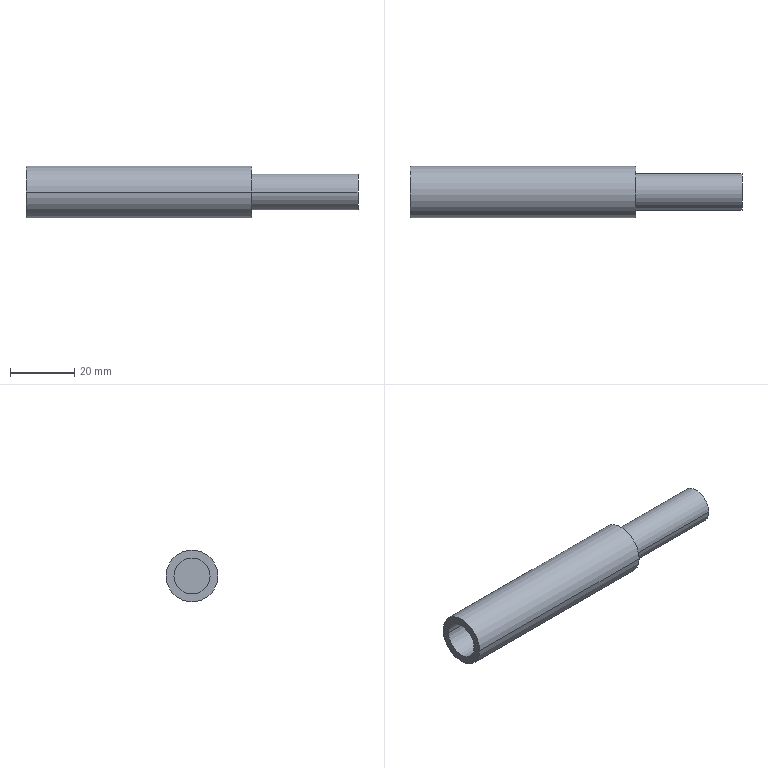Component | SolidWorks | MotorAxisHousing3-1 | 1 solid | 10 faces | box 103 x 16 x 16 mm | volume 12399 mm3 | cylinder 6 | plane 4 | commonest cylinder face diameters 11.2 x4 16 x2
build123d program:
from build123d import *

# Parameters (mm, degrees)
BOSS_EXTRUDE1_DEPTH      = 10
BOSS_EXTRUDE1_DEPTH_BACK = 43
SKETCH1_R                = 5.6
BOSS_EXTRUDE2_DEPTH      = 50
BOSS_EXTRUDE2_DEPTH_BACK = 20
SKETCH2_R                = 8
SKETCH2_R_2              = 5.6


with BuildPart() as part:
    # Sketch1 → Boss-Extrude1 (new, two sides: drawn at the far end of the back side and taken through both)
    with BuildSketch(Plane.XY.offset(-BOSS_EXTRUDE1_DEPTH_BACK)):
        with Locations((92, 0)):
            Circle(SKETCH1_R)
    extrude(amount=BOSS_EXTRUDE1_DEPTH + BOSS_EXTRUDE1_DEPTH_BACK)

    # Sketch2 → Boss-Extrude2 (add, two sides: drawn at the far end of the back side and taken through both)
    with BuildSketch(Plane.XY.offset(10).offset(-BOSS_EXTRUDE2_DEPTH_BACK)):
        with Locations((92, 0)):
            Circle(SKETCH2_R)
        with Locations((92, 0)):
            Circle(SKETCH2_R_2, mode=Mode.SUBTRACT)
    extrude(amount=BOSS_EXTRUDE2_DEPTH + BOSS_EXTRUDE2_DEPTH_BACK)


solid = part.part

# Placed as in the assembly
solid = solid.moved(Location((-500, 92, -92), (0, -90, 0)))
STEP:
#1=COLOUR_RGB('',0.7922,0.8196,0.9333);
#2=FILL_AREA_STYLE_COLOUR('',#1);
#3=FILL_AREA_STYLE('',(#2));
#4=SURFACE_STYLE_FILL_AREA(#3);
#5=SURFACE_SIDE_STYLE('',(#4));
#6=SURFACE_STYLE_USAGE(.BOTH.,#5);
#7=PRESENTATION_STYLE_ASSIGNMENT((#6));
#8=CARTESIAN_POINT('',(-20.079,3.402,0.));
#9=VERTEX_POINT('',#8);
#10=CARTESIAN_POINT('',(-20.079,3.843,0.));
#11=VERTEX_POINT('',#10);
#12=CARTESIAN_POINT('',(-20.079,3.622,0.));
#13=DIRECTION('',(-1.,0.,0.));
#14=DIRECTION('',(0.,1.,0.));
#15=AXIS2_PLACEMENT_3D('',#12,#13,#14);
#16=CIRCLE('',#15,0.2205);
#17=EDGE_CURVE('',#9,#11,#16,.T.);
#18=ORIENTED_EDGE('',*,*,#17,.F.);
#19=CARTESIAN_POINT('',(-22.047,3.402,0.));
#20=VERTEX_POINT('',#19);
#21=CARTESIAN_POINT('',(-19.291,3.402,0.));
#22=DIRECTION('',(-1.,0.,0.));
#23=VECTOR('',#22,39.37);
#24=LINE('',#21,#23);
#25=EDGE_CURVE('',#9,#20,#24,.T.);
#26=ORIENTED_EDGE('',*,*,#25,.T.);
#27=CARTESIAN_POINT('',(-22.047,3.843,0.));
#28=VERTEX_POINT('',#27);
#29=CARTESIAN_POINT('',(-22.047,3.622,0.));
#30=DIRECTION('',(-1.,0.,0.));
#31=DIRECTION('',(0.,1.,0.));
#32=AXIS2_PLACEMENT_3D('',#29,#30,#31);
#33=CIRCLE('',#32,0.2205);
#34=EDGE_CURVE('',#20,#28,#33,.T.);
#35=ORIENTED_EDGE('',*,*,#34,.T.);
#36=CARTESIAN_POINT('',(-19.291,3.843,0.));
#37=DIRECTION('',(-1.,0.,0.));
#38=VECTOR('',#37,39.37);
#39=LINE('',#36,#38);
#40=EDGE_CURVE('',#11,#28,#39,.T.);
#41=ORIENTED_EDGE('',*,*,#40,.F.);
#42=EDGE_LOOP('',(#18,#26,#35,#41));
#43=FACE_OUTER_BOUND('',#42,.T.);
#44=CARTESIAN_POINT('',(-19.291,3.622,0.));
#45=DIRECTION('',(-1.,0.,0.));
#46=DIRECTION('',(0.,1.,0.));
#47=AXIS2_PLACEMENT_3D('',#44,#45,#46);
#48=CYLINDRICAL_SURFACE('',#47,0.2205);
#49=ADVANCED_FACE('',(#43),#48,.F.);
#50=CARTESIAN_POINT('',(-19.291,3.937,0.));
#51=VERTEX_POINT('',#50);
#52=CARTESIAN_POINT('',(-19.291,3.307,0.));
#53=VERTEX_POINT('',#52);
#54=CARTESIAN_POINT('',(-19.291,3.622,0.));
#55=DIRECTION('',(-1.,0.,0.));
#56=DIRECTION('',(0.,1.,0.));
#57=AXIS2_PLACEMENT_3D('',#54,#55,#56);
#58=CIRCLE('',#57,0.315);
#59=EDGE_CURVE('',#51,#53,#58,.T.);
#60=ORIENTED_EDGE('',*,*,#59,.T.);
#61=CARTESIAN_POINT('',(-22.047,3.307,0.));
#62=VERTEX_POINT('',#61);
#63=CARTESIAN_POINT('',(-19.291,3.307,0.));
#64=DIRECTION('',(-1.,0.,0.));
#65=VECTOR('',#64,39.37);
#66=LINE('',#63,#65);
#67=EDGE_CURVE('',#53,#62,#66,.T.);
#68=ORIENTED_EDGE('',*,*,#67,.T.);
#69=CARTESIAN_POINT('',(-22.047,3.937,0.));
#70=VERTEX_POINT('',#69);
#71=CARTESIAN_POINT('',(-22.047,3.622,0.));
#72=DIRECTION('',(-1.,0.,0.));
#73=DIRECTION('',(0.,1.,0.));
#74=AXIS2_PLACEMENT_3D('',#71,#72,#73);
#75=CIRCLE('',#74,0.315);
#76=EDGE_CURVE('',#70,#62,#75,.T.);
#77=ORIENTED_EDGE('',*,*,#76,.F.);
#78=CARTESIAN_POINT('',(-19.291,3.937,0.));
#79=DIRECTION('',(-1.,0.,0.));
#80=VECTOR('',#79,39.37);
#81=LINE('',#78,#80);
#82=EDGE_CURVE('',#51,#70,#81,.T.);
#83=ORIENTED_EDGE('',*,*,#82,.F.);
#84=EDGE_LOOP('',(#60,#68,#77,#83));
#85=FACE_OUTER_BOUND('',#84,.T.);
#86=CARTESIAN_POINT('',(-19.291,3.622,0.));
#87=DIRECTION('',(-1.,0.,0.));
#88=DIRECTION('',(0.,1.,0.));
#89=AXIS2_PLACEMENT_3D('',#86,#87,#88);
#90=CYLINDRICAL_SURFACE('',#89,0.315);
#91=ADVANCED_FACE('',(#85),#90,.T.);
#92=CARTESIAN_POINT('',(-19.291,3.843,0.));
#93=VERTEX_POINT('',#92);
#94=CARTESIAN_POINT('',(-19.291,3.402,0.));
#95=VERTEX_POINT('',#94);
#96=CARTESIAN_POINT('',(-19.291,3.622,0.));
#97=DIRECTION('',(-1.,0.,0.));
#98=DIRECTION('',(0.,1.,0.));
#99=AXIS2_PLACEMENT_3D('',#96,#97,#98);
#100=CIRCLE('',#99,0.2205);
#101=EDGE_CURVE('',#93,#95,#100,.T.);
#102=ORIENTED_EDGE('',*,*,#101,.F.);
#103=CARTESIAN_POINT('',(-17.992,3.843,0.));
#104=VERTEX_POINT('',#103);
#105=CARTESIAN_POINT('',(-20.079,3.843,0.));
#106=DIRECTION('',(1.,0.,0.));
#107=VECTOR('',#106,39.37);
#108=LINE('',#105,#107);
#109=EDGE_CURVE('',#93,#104,#108,.T.);
#110=ORIENTED_EDGE('',*,*,#109,.T.);
#111=CARTESIAN_POINT('',(-17.992,3.402,0.));
#112=VERTEX_POINT('',#111);
#113=CARTESIAN_POINT('',(-17.992,3.622,0.));
#114=DIRECTION('',(-1.,0.,0.));
#115=DIRECTION('',(0.,1.,0.));
#116=AXIS2_PLACEMENT_3D('',#113,#114,#115);
#117=CIRCLE('',#116,0.2205);
#118=EDGE_CURVE('',#104,#112,#117,.T.);
#119=ORIENTED_EDGE('',*,*,#118,.T.);
#120=CARTESIAN_POINT('',(-20.079,3.402,0.));
#121=DIRECTION('',(1.,0.,0.));
#122=VECTOR('',#121,39.37);
#123=LINE('',#120,#122);
#124=EDGE_CURVE('',#95,#112,#123,.T.);
#125=ORIENTED_EDGE('',*,*,#124,.F.);
#126=EDGE_LOOP('',(#102,#110,#119,#125));
#127=FACE_OUTER_BOUND('',#126,.T.);
#128=CARTESIAN_POINT('',(-20.079,3.622,0.));
#129=DIRECTION('',(1.,0.,0.));
#130=DIRECTION('',(0.,-1.,0.));
#131=AXIS2_PLACEMENT_3D('',#128,#129,#130);
#132=CYLINDRICAL_SURFACE('',#131,0.2205);
#133=ADVANCED_FACE('',(#127),#132,.T.);
#134=ORIENTED_EDGE('',*,*,#109,.F.);
#135=CARTESIAN_POINT('',(-19.291,3.622,0.));
#136=DIRECTION('',(-1.,0.,0.));
#137=DIRECTION('',(0.,1.,0.));
#138=AXIS2_PLACEMENT_3D('',#135,#136,#137);
#139=CIRCLE('',#138,0.2205);
#140=EDGE_CURVE('',#95,#93,#139,.T.);
#141=ORIENTED_EDGE('',*,*,#140,.F.);
#142=ORIENTED_EDGE('',*,*,#124,.T.);
#143=CARTESIAN_POINT('',(-17.992,3.622,0.));
#144=DIRECTION('',(-1.,0.,0.));
#145=DIRECTION('',(0.,1.,0.));
#146=AXIS2_PLACEMENT_3D('',#143,#144,#145);
#147=CIRCLE('',#146,0.2205);
#148=EDGE_CURVE('',#112,#104,#147,.T.);
#149=ORIENTED_EDGE('',*,*,#148,.T.);
#150=EDGE_LOOP('',(#134,#141,#142,#149));
#151=FACE_OUTER_BOUND('',#150,.T.);
#152=CARTESIAN_POINT('',(-20.079,3.622,0.));
#153=DIRECTION('',(1.,0.,0.));
#154=DIRECTION('',(0.,-1.,0.));
#155=AXIS2_PLACEMENT_3D('',#152,#153,#154);
#156=CYLINDRICAL_SURFACE('',#155,0.2205);
#157=ADVANCED_FACE('',(#151),#156,.T.);
#158=ORIENTED_EDGE('',*,*,#148,.F.);
#159=ORIENTED_EDGE('',*,*,#118,.F.);
#160=EDGE_LOOP('',(#158,#159));
#161=FACE_OUTER_BOUND('',#160,.T.);
#162=CARTESIAN_POINT('',(-17.992,3.622,0.));
#163=DIRECTION('',(-1.,0.,0.));
#164=DIRECTION('',(0.,1.,0.));
#165=AXIS2_PLACEMENT_3D('',#162,#163,#164);
#166=PLANE('',#165);
#167=ADVANCED_FACE('',(#161),#166,.F.);
#168=ORIENTED_EDGE('',*,*,#67,.F.);
#169=CARTESIAN_POINT('',(-19.291,3.622,0.));
#170=DIRECTION('',(-1.,0.,0.));
#171=DIRECTION('',(0.,1.,0.));
#172=AXIS2_PLACEMENT_3D('',#169,#170,#171);
#173=CIRCLE('',#172,0.315);
#174=EDGE_CURVE('',#53,#51,#173,.T.);
#175=ORIENTED_EDGE('',*,*,#174,.T.);
#176=ORIENTED_EDGE('',*,*,#82,.T.);
#177=CARTESIAN_POINT('',(-22.047,3.622,0.));
#178=DIRECTION('',(-1.,0.,0.));
#179=DIRECTION('',(0.,1.,0.));
#180=AXIS2_PLACEMENT_3D('',#177,#178,#179);
#181=CIRCLE('',#180,0.315);
#182=EDGE_CURVE('',#62,#70,#181,.T.);
#183=ORIENTED_EDGE('',*,*,#182,.F.);
#184=EDGE_LOOP('',(#168,#175,#176,#183));
#185=FACE_OUTER_BOUND('',#184,.T.);
#186=CARTESIAN_POINT('',(-19.291,3.622,0.));
#187=DIRECTION('',(-1.,0.,0.));
#188=DIRECTION('',(0.,1.,0.));
#189=AXIS2_PLACEMENT_3D('',#186,#187,#188);
#190=CYLINDRICAL_SURFACE('',#189,0.315);
#191=ADVANCED_FACE('',(#185),#190,.T.);
#192=ORIENTED_EDGE('',*,*,#140,.T.);
#193=ORIENTED_EDGE('',*,*,#101,.T.);
#194=EDGE_LOOP('',(#192,#193));
#195=FACE_BOUND('',#194,.T.);
#196=ORIENTED_EDGE('',*,*,#59,.F.);
#197=ORIENTED_EDGE('',*,*,#174,.F.);
#198=EDGE_LOOP('',(#196,#197));
#199=FACE_OUTER_BOUND('',#198,.T.);
#200=CARTESIAN_POINT('',(-19.291,3.622,0.));
#201=DIRECTION('',(-1.,0.,0.));
#202=DIRECTION('',(0.,1.,0.));
#203=AXIS2_PLACEMENT_3D('',#200,#201,#202);
#204=PLANE('',#203);
#205=ADVANCED_FACE('',(#195,#199),#204,.F.);
#206=ORIENTED_EDGE('',*,*,#25,.F.);
#207=CARTESIAN_POINT('',(-20.079,3.622,0.));
#208=DIRECTION('',(-1.,0.,0.));
#209=DIRECTION('',(0.,1.,0.));
#210=AXIS2_PLACEMENT_3D('',#207,#208,#209);
#211=CIRCLE('',#210,0.2205);
#212=EDGE_CURVE('',#11,#9,#211,.T.);
#213=ORIENTED_EDGE('',*,*,#212,.F.);
#214=ORIENTED_EDGE('',*,*,#40,.T.);
#215=CARTESIAN_POINT('',(-22.047,3.622,0.));
#216=DIRECTION('',(-1.,0.,0.));
#217=DIRECTION('',(0.,1.,0.));
#218=AXIS2_PLACEMENT_3D('',#215,#216,#217);
#219=CIRCLE('',#218,0.2205);
#220=EDGE_CURVE('',#28,#20,#219,.T.);
#221=ORIENTED_EDGE('',*,*,#220,.T.);
#222=EDGE_LOOP('',(#206,#213,#214,#221));
#223=FACE_OUTER_BOUND('',#222,.T.);
#224=CARTESIAN_POINT('',(-19.291,3.622,0.));
#225=DIRECTION('',(-1.,0.,0.));
#226=DIRECTION('',(0.,1.,0.));
#227=AXIS2_PLACEMENT_3D('',#224,#225,#226);
#228=CYLINDRICAL_SURFACE('',#227,0.2205);
#229=ADVANCED_FACE('',(#223),#228,.F.);
#230=ORIENTED_EDGE('',*,*,#76,.T.);
#231=ORIENTED_EDGE('',*,*,#182,.T.);
#232=EDGE_LOOP('',(#230,#231));
#233=FACE_OUTER_BOUND('',#232,.T.);
#234=ORIENTED_EDGE('',*,*,#220,.F.);
#235=ORIENTED_EDGE('',*,*,#34,.F.);
#236=EDGE_LOOP('',(#234,#235));
#237=FACE_BOUND('',#236,.T.);
#238=CARTESIAN_POINT('',(-22.047,3.622,0.));
#239=DIRECTION('',(-1.,0.,0.));
#240=DIRECTION('',(0.,1.,0.));
#241=AXIS2_PLACEMENT_3D('',#238,#239,#240);
#242=PLANE('',#241);
#243=ADVANCED_FACE('',(#233,#237),#242,.T.);
#244=ORIENTED_EDGE('',*,*,#212,.T.);
#245=ORIENTED_EDGE('',*,*,#17,.T.);
#246=EDGE_LOOP('',(#244,#245));
#247=FACE_OUTER_BOUND('',#246,.T.);
#248=CARTESIAN_POINT('',(-20.079,3.622,0.));
#249=DIRECTION('',(-1.,0.,0.));
#250=DIRECTION('',(0.,1.,0.));
#251=AXIS2_PLACEMENT_3D('',#248,#249,#250);
#252=PLANE('',#251);
#253=ADVANCED_FACE('',(#247),#252,.T.);
#254=CLOSED_SHELL('',(#49,#91,#133,#157,#167,#191,#205,#229,#243,#253));
#255=MANIFOLD_SOLID_BREP('',#254);
#256=STYLED_ITEM('',(#7),#255);
#257=(LENGTH_UNIT()NAMED_UNIT(*)SI_UNIT($,.METRE.));
#258=LENGTH_MEASURE_WITH_UNIT(LENGTH_MEASURE(0.0254),#257);
#259=DIMENSIONAL_EXPONENTS(1.,0.,0.,0.,0.,0.,0.);
#260=(CONVERSION_BASED_UNIT('',#258)LENGTH_UNIT()NAMED_UNIT(#259));
#261=UNCERTAINTY_MEASURE_WITH_UNIT(LENGTH_MEASURE(0.00001),#260,'','');
#262=(NAMED_UNIT(*)PLANE_ANGLE_UNIT()SI_UNIT($,.RADIAN.));
#263=(NAMED_UNIT(*)SI_UNIT($,.STERADIAN.)SOLID_ANGLE_UNIT());
#264=(GEOMETRIC_REPRESENTATION_CONTEXT(3)GLOBAL_UNCERTAINTY_ASSIGNED_CONTEXT((#261))GLOBAL_UNIT_ASSIGNED_CONTEXT((#260,#262,#263))REPRESENTATION_CONTEXT('',''));
#265=MECHANICAL_DESIGN_GEOMETRIC_PRESENTATION_REPRESENTATION('',(#256),#264);
#266=PRESENTATION_LAYER_ASSIGNMENT('','',(#256));
#267=CARTESIAN_POINT('',(0.,0.,0.));
#268=DIRECTION('',(0.,0.,1.));
#269=DIRECTION('',(1.,0.,0.));
#270=AXIS2_PLACEMENT_3D('',#267,#268,#269);
#271=(LENGTH_UNIT()NAMED_UNIT(*)SI_UNIT($,.METRE.));
#272=LENGTH_MEASURE_WITH_UNIT(LENGTH_MEASURE(0.0254),#271);
#273=DIMENSIONAL_EXPONENTS(1.,0.,0.,0.,0.,0.,0.);
#274=(CONVERSION_BASED_UNIT('',#272)LENGTH_UNIT()NAMED_UNIT(#273));
#275=UNCERTAINTY_MEASURE_WITH_UNIT(LENGTH_MEASURE(0.00001),#274,'','');
#276=(NAMED_UNIT(*)PLANE_ANGLE_UNIT()SI_UNIT($,.RADIAN.));
#277=(NAMED_UNIT(*)SI_UNIT($,.STERADIAN.)SOLID_ANGLE_UNIT());
#278=(GEOMETRIC_REPRESENTATION_CONTEXT(3)GLOBAL_UNCERTAINTY_ASSIGNED_CONTEXT((#275))GLOBAL_UNIT_ASSIGNED_CONTEXT((#274,#276,#277))REPRESENTATION_CONTEXT('',''));
#279=ADVANCED_BREP_SHAPE_REPRESENTATION('',(#255,#270),#278);